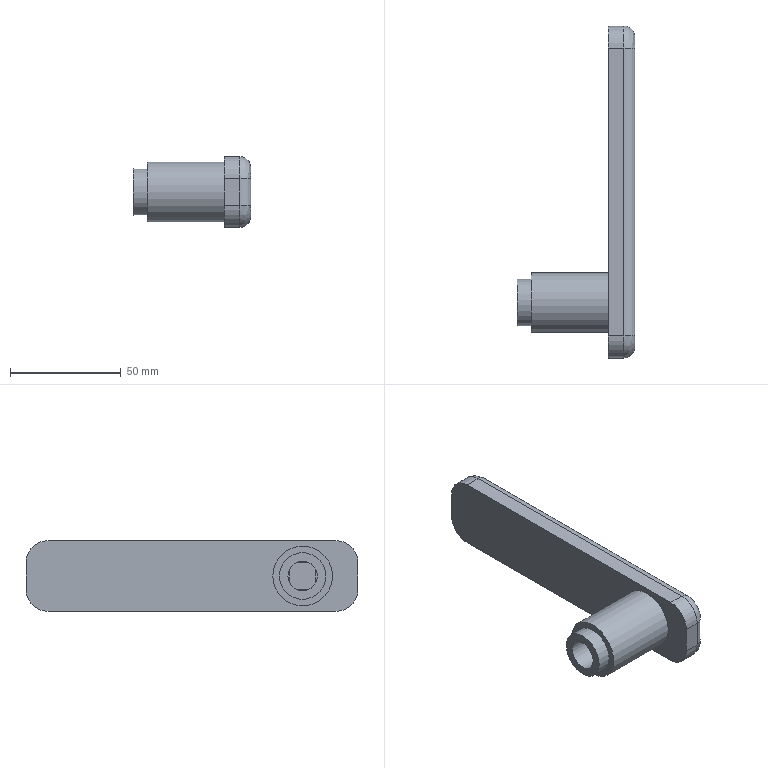Component | NX | HANDLE | 1 solid | 32 faces | volume 73464 mm3 | plane 17 | cylinder 11 | spline 4 | commonest cylinder face diameters 20 x4 10 x4 13.3 x1 27 x1 21 x1